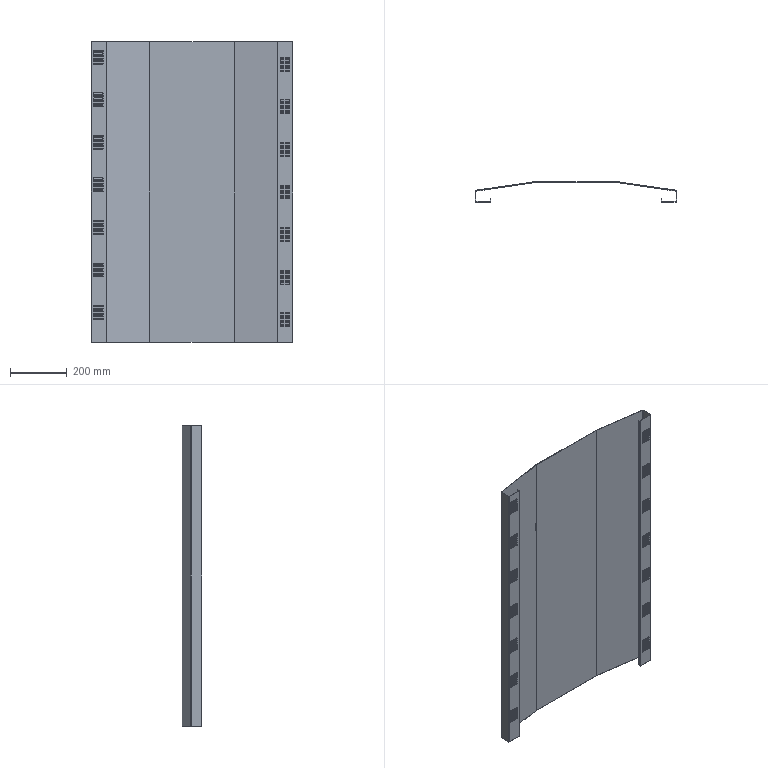Component | SolidWorks | TopCover01100-2_TopCover01100-1 | 1 solid | 494 faces | volume 1433406 mm3 | cylinder 268 | plane 226 | commonest cylinder face diameters 4 x252 4.473 x8 1.473 x8